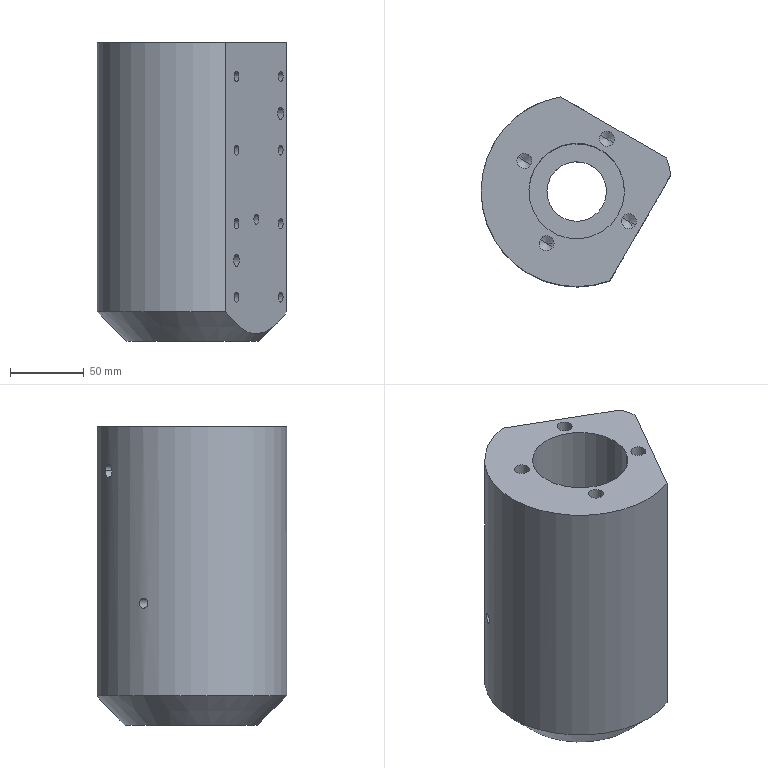Component | SolidWorks | KLHFH003PinSlider-SymmetricPart(2)-1 | 1 solid | 115 faces | box 129.07 x 129.07 x 203 mm | volume 1659462 mm3 | cylinder 60 | cone 50 | plane 5 | commonest cylinder face diameters 6.8 x36 8 x8 10.2 x8 8.8 x2 65 x2 40.5 x2 130 x2 | material Plain Carbon Steel
build123d program:
from build123d import *

# Parameters (mm, degrees)
SKETCH1_R                       = 65
BOSS_EXTRUDE1_DEPTH             = 101.5
CHAMFER1_SIZE                   = 20
SKETCH2_W                       = 83.066
SKETCH2_H                       = 30
CUT_EXTRUDE2_DEPTH              = 223.843
CIRPATTERN1_COUNT               = 2
CIRPATTERN1_ANGLE               = 90
SKETCH3_R                       = 20.25
CUT_EXTRUDE3_DEPTH              = 80
SKETCH4_R                       = 20.25
CUT_EXTRUDE4_DEPTH              = 154.555
SKETCH5_R                       = 32.5
CUT_EXTRUDE5_DEPTH              = 170
M8_TAPPED_HOLE1_D               = 6.8
M8_TAPPED_HOLE1_DEPTH           = 22.25
M8_TAPPED_HOLE1_TIP             = 2.043
M8_TAPPED_HOLE2_D               = 6.8
M8_TAPPED_HOLE2_DEPTH           = 22.25
M8_TAPPED_HOLE2_TIP             = 2.043
CIRPATTERN2_COUNT               = 4
G1_8_TAPPED_HOLE1_D             = 8.8
G1_8_TAPPED_HOLE1_DEPTH         = 50
G1_8_TAPPED_HOLE1_TIP           = 2.644
SIZE_MM_DOWEL_PIN_HOLE2_D       = 8
SIZE_MM_DOWEL_PIN_HOLE2_DEPTH   = 15
SIZE_MM_DOWEL_PIN_HOLE2_TIP     = 2.403
SIZE_MM_DOWEL_PIN_HOLE2_2_D     = 8
SIZE_MM_DOWEL_PIN_HOLE2_2_DEPTH = 15
SIZE_MM_DOWEL_PIN_HOLE2_2_TIP   = 2.403
M8_TAPPED_HOLE3_D               = 6.8


with BuildPart() as part:
    # Sketch1 → Boss-Extrude1 (new, symmetric)
    with BuildSketch(Plane.XY):
        with Locations(Location((0, 0, 0), (0, 0, 180))):
            Circle(SKETCH1_R)
    extrude(amount=BOSS_EXTRUDE1_DEPTH, both=True)

    # Chamfer1
    chamfer1_edges = [part.edges().sort_by_distance(p)[0] for p in [
        (65, 0, 101.5),
    ]]
    chamfer(chamfer1_edges, length=CHAMFER1_SIZE)

    # Sketch2 → Cut-Extrude2 (cut, through all)
    with BuildSketch(Plane.XY.offset(101.5)):
        with Locations((0, 65)):
            Rectangle(SKETCH2_W, SKETCH2_H)
    cut_extrude2 = extrude(amount=-CUT_EXTRUDE2_DEPTH, mode=Mode.SUBTRACT)

    # CirPattern1: Cut-Extrude2 ×2 about axis
    cirpattern1_axis = Axis((0, 0, 101.5), (0, 0, 1))
    for i in range(1, CIRPATTERN1_COUNT):
        add(cut_extrude2.rotate(cirpattern1_axis, i * CIRPATTERN1_ANGLE / (CIRPATTERN1_COUNT - 1)), mode=Mode.SUBTRACT)

    # Sketch3 → Cut-Extrude3 (cut)
    with BuildSketch(Plane.XY.offset(101.5)):
        Circle(SKETCH3_R)
    extrude(amount=-CUT_EXTRUDE3_DEPTH, mode=Mode.SUBTRACT)

    # Sketch4 → Cut-Extrude4 (cut, through all)
    with BuildSketch(Plane.XY.offset(21.5)):
        Circle(SKETCH4_R)
    extrude(amount=-CUT_EXTRUDE4_DEPTH, mode=Mode.SUBTRACT)

    # Sketch5 → Cut-Extrude5 (cut)
    with BuildSketch(Plane(origin=(0, 0, -101.5), x_dir=(-1, 0, 0), z_dir=(0, 0, -1))):
        Circle(SKETCH5_R)
    extrude(amount=-CUT_EXTRUDE5_DEPTH, mode=Mode.SUBTRACT)

    # M8 Tapped Hole1
    with Locations(Plane(origin=(0, 50, 0), x_dir=(1, 0, 0), z_dir=(0, 1, 0))):
        with Locations((-33, 88.5), (27, 88.5), (-33, 38.5), (27, 38.5), (-33, -11.5), (27, -11.5), (-33, -61.5), (27, -61.5)):
            Hole(M8_TAPPED_HOLE1_D / 2, depth=M8_TAPPED_HOLE1_DEPTH)
            with Locations((0, 0, -(M8_TAPPED_HOLE1_DEPTH + M8_TAPPED_HOLE1_TIP / 2))):  # 118° drill point
                Cone(0, M8_TAPPED_HOLE1_D / 2, M8_TAPPED_HOLE1_TIP, mode=Mode.SUBTRACT)

    # M8 Tapped Hole2
    with Locations(Plane.ZY.offset(50)):
        with Locations((-78.5, 33), (-28.5, 33), (21.5, 33), (71.5, 33), (-78.5, -27), (-28.5, -27), (21.5, -27), (71.5, -27)):
            Hole(M8_TAPPED_HOLE2_D / 2, depth=M8_TAPPED_HOLE2_DEPTH)
            with Locations((0, 0, -(M8_TAPPED_HOLE2_DEPTH + M8_TAPPED_HOLE2_TIP / 2))):  # 118° drill point
                Cone(0, M8_TAPPED_HOLE2_D / 2, M8_TAPPED_HOLE2_TIP, mode=Mode.SUBTRACT)

    # Sketch10 → M12 Tapped Hole1 (revolve, cut)
    with BuildSketch(Plane(origin=(41, 0, -101.5), x_dir=(0, 1, 0), z_dir=(1, 0, 0))):
        Polygon((0, 0), (0, 41.814), (5.1, 38.75), (5.1, 0), align=None)
    m12_tapped_hole1 = revolve(axis=Axis((41, 0, -107.85), (0, 0, 1)), mode=Mode.SUBTRACT)

    # CirPattern2: M12 Tapped Hole1 ×4 about axis
    cirpattern2_axis = Axis((0, 0, 0), (0, 0, 1))
    for i in range(1, CIRPATTERN2_COUNT):
        add(m12_tapped_hole1.rotate(cirpattern2_axis, i * 360 / CIRPATTERN2_COUNT), mode=Mode.SUBTRACT)

    # G1_8 Tapped Hole1
    with Locations(Plane(origin=(56.292, 32.5, 0), x_dir=(0, 0, -1), z_dir=(0.866, 0.5, 0))):
        with Locations((71.5, 0)):
            Hole(G1_8_TAPPED_HOLE1_D / 2, depth=G1_8_TAPPED_HOLE1_DEPTH)
            with Locations((0, 0, -(G1_8_TAPPED_HOLE1_DEPTH + G1_8_TAPPED_HOLE1_TIP / 2))):  # 118° drill point
                Cone(0, G1_8_TAPPED_HOLE1_D / 2, G1_8_TAPPED_HOLE1_TIP, mode=Mode.SUBTRACT)

    # Size mm Dowel Pin Hole2
    with Locations(Plane(origin=(0, 50, 0), x_dir=(1, 0, 0), z_dir=(0, 1, 0))):
        with Locations((-33, -36.5), (27, 63.5)):
            Hole(SIZE_MM_DOWEL_PIN_HOLE2_D / 2, depth=SIZE_MM_DOWEL_PIN_HOLE2_DEPTH)
            with Locations((0, 0, -(SIZE_MM_DOWEL_PIN_HOLE2_DEPTH + SIZE_MM_DOWEL_PIN_HOLE2_TIP / 2))):  # 118° drill point
                Cone(0, SIZE_MM_DOWEL_PIN_HOLE2_D / 2, SIZE_MM_DOWEL_PIN_HOLE2_TIP, mode=Mode.SUBTRACT)

    # Size mm Dowel Pin Hole2_2
    with Locations(Plane.ZY.offset(50)):
        with Locations((-53.5, 33), (46.5, -27)):
            Hole(SIZE_MM_DOWEL_PIN_HOLE2_2_D / 2, depth=SIZE_MM_DOWEL_PIN_HOLE2_2_DEPTH)
            with Locations((0, 0, -(SIZE_MM_DOWEL_PIN_HOLE2_2_DEPTH + SIZE_MM_DOWEL_PIN_HOLE2_2_TIP / 2))):  # 118° drill point
                Cone(0, SIZE_MM_DOWEL_PIN_HOLE2_2_D / 2, SIZE_MM_DOWEL_PIN_HOLE2_2_TIP, mode=Mode.SUBTRACT)

    # M8 Tapped Hole3 (through all)
    with Locations(Plane.ZY.offset(50)):
        with Locations((18.5, 0)):
            Hole(M8_TAPPED_HOLE3_D / 2)


solid = part.part

# Placed as in the assembly
solid = solid.moved(Location((91, 157.617, -276), (180, -0.0001762, -150)))